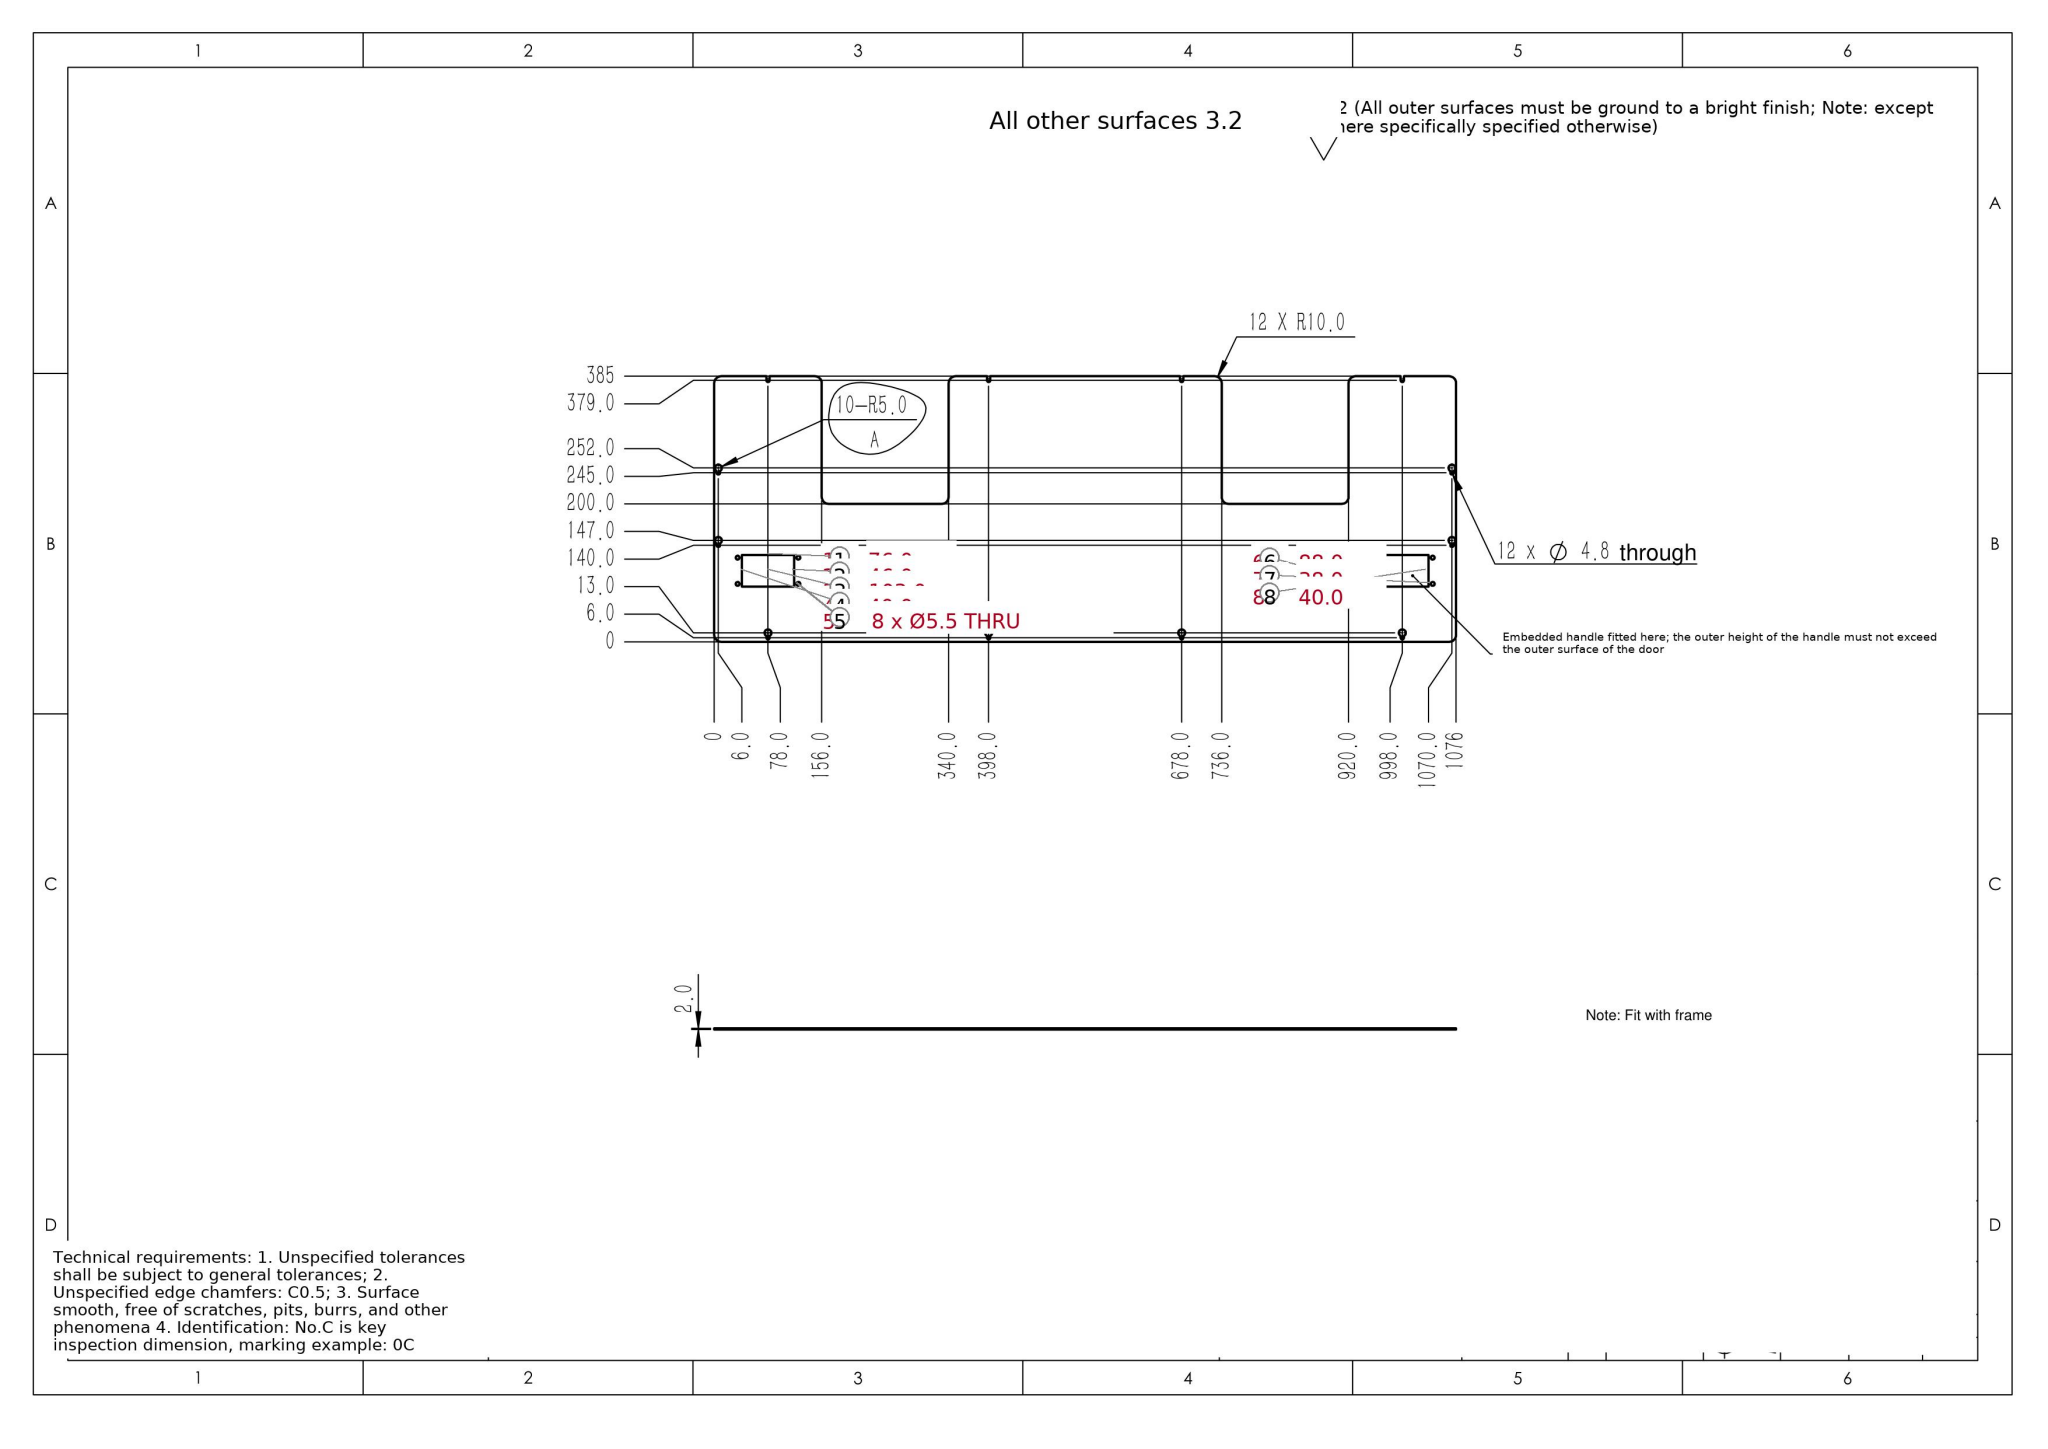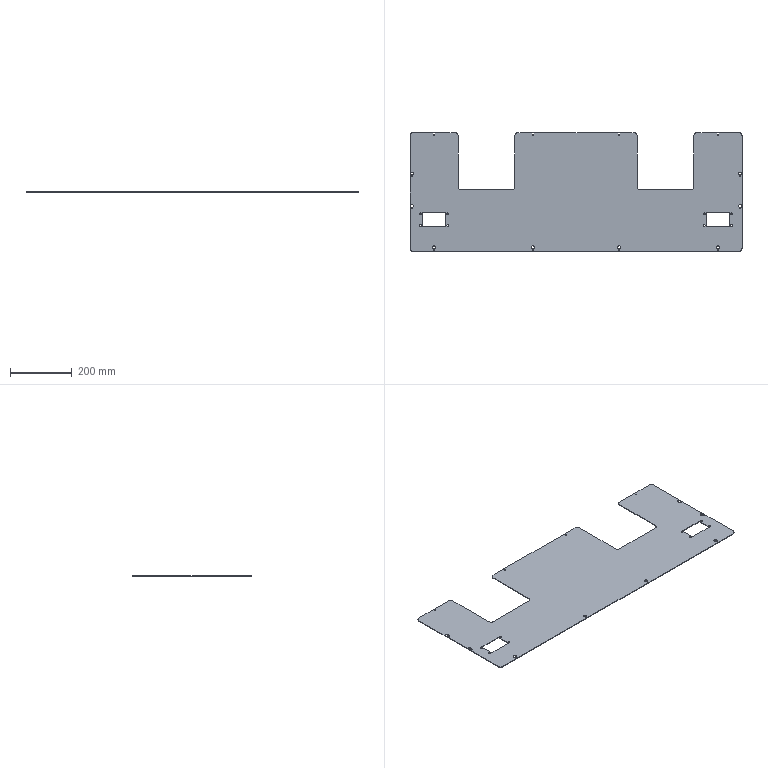Part | SolidWorks | mm | 1 solid | 114 faces | box 1076 x 385 x 2 mm | volume 675951 mm3 | cylinder 64 | plane 50 | commonest cylinder face diameters 10 x24 5.5 x16 20 x12 4.8 x12
build123d program:
from build123d import *

# Parameters (mm, degrees)
SKETCH1_W                      = 1076
SKETCH1_H                      = 385
BOSS_EXTRUDE1_DEPTH            = 2
SKETCH2_W                      = 184
SKETCH2_H                      = 185
CUT_EXTRUDE1_DEPTH             = 2
FILLET1_R                      = 10
F_4_8_4_8_DIAMETER_HOLE1_D     = 4.8
SKETCH5_W                      = 76
SKETCH5_H                      = 46
CUT_EXTRUDE2_DEPTH             = 10
F_5_5_5_5_DIAMETER_HOLE1_D     = 5.5
F_5_5_5_5_DIAMETER_HOLE1_DEPTH = 2
F_5_5_5_5_DIAMETER_HOLE1_TIP   = 1.652
CUT_EXTRUDE3_DEPTH             = 10
SKETCH11_W                     = 4.8
SKETCH11_H                     = 6
CUT_EXTRUDE4_DEPTH             = 10


with BuildPart() as part:
    # Sketch1 → Boss-Extrude1 (new body)
    with BuildSketch(Plane.XY):
        Rectangle(SKETCH1_W, SKETCH1_H)
    extrude(amount=BOSS_EXTRUDE1_DEPTH)

    # Sketch2 → Cut-Extrude1 (cut)
    with BuildSketch(Plane.XY.offset(2)):
        with Locations((-290, 100)):
            Rectangle(SKETCH2_W, SKETCH2_H)
        with Locations((290, 100)):
            Rectangle(SKETCH2_W, SKETCH2_H)
    extrude(amount=-CUT_EXTRUDE1_DEPTH, mode=Mode.SUBTRACT)

    # Fillet1
    fillet1_edges = [part.edges().sort_by_distance(p)[0] for p in [
        (-382, 7.5, 1),
        (-382, 192.5, 1),
        (-198, 192.5, 1),
        (-198, 7.5, 1),
        (198, 7.5, 1),
        (198, 192.5, 1),
        (382, 192.5, 1),
        (382, 7.5, 1),
        (538, -192.5, 1),
        (-538, -192.5, 1),
        (-538, 192.5, 1),
        (538, 192.5, 1),
    ]]
    fillet(fillet1_edges, radius=FILLET1_R)

    # 4.8 _4.8_ Diameter Hole1 (through all)
    with Locations(Plane(origin=(0, 0, 0), x_dir=(-1, 0, 0), z_dir=(0, 0, -1))):
        with Locations((-140, 186.5), (140, 186.5), (460, 186.5), (-460, 186.5), (-532, 52.5), (532, 52.5), (532, -52.5), (460, -186.5), (140, -186.5), (-140, -186.5), (-460, -186.5), (-532, -52.5)):
            Hole(F_4_8_4_8_DIAMETER_HOLE1_D / 2)

    # Sketch5 → Cut-Extrude2 (cut)
    with BuildSketch(Plane(origin=(0, 0, 0), x_dir=(-1, 0, 0), z_dir=(0, 0, -1))):
        with Locations((-460, -89.5)):
            Rectangle(SKETCH5_W, SKETCH5_H)
        with Locations((460, -89.5)):
            Rectangle(SKETCH5_W, SKETCH5_H)
    extrude(amount=-CUT_EXTRUDE2_DEPTH, mode=Mode.SUBTRACT)

    # 5.5 _5.5_ Diameter Hole1
    with Locations(Plane(origin=(0, 0, 0), x_dir=(-1, 0, 0), z_dir=(0, 0, -1))):
        with Locations((504, -108.5), (416, -108.5), (504, -70.5), (416, -70.5), (-416, -70.5), (-416, -108.5), (-504, -70.5), (-504, -108.5)):
            Hole(F_5_5_5_5_DIAMETER_HOLE1_D / 2, depth=F_5_5_5_5_DIAMETER_HOLE1_DEPTH)
            with Locations((0, 0, -(F_5_5_5_5_DIAMETER_HOLE1_DEPTH + F_5_5_5_5_DIAMETER_HOLE1_TIP / 2))):  # 118° drill point
                Cone(0, F_5_5_5_5_DIAMETER_HOLE1_D / 2, F_5_5_5_5_DIAMETER_HOLE1_TIP, mode=Mode.SUBTRACT)

    # Sketch10 → Cut-Extrude3 (cut)
    with BuildSketch(Plane.XY.offset(2)):
        with BuildLine():
            Line((462.4, -186.5), (462.4, -183.886))
            ThreePointArc((462.4, -183.886), (460, -174.5), (457.6, -183.886))
            Line((457.6, -183.886), (457.6, -186.5))
            Line((457.6, -186.5), (462.4, -186.5))
        make_face()
        with BuildLine():
            Line((142.4, -186.5), (137.6, -186.5))
            Line((137.6, -186.5), (137.6, -183.886))
            ThreePointArc((137.6, -183.886), (140, -174.5), (142.4, -183.886))
            Line((142.4, -183.886), (142.4, -186.5))
        make_face()
        with BuildLine():
            Line((-142.4, -186.5), (-142.4, -183.886))
            ThreePointArc((-142.4, -183.886), (-140, -174.5), (-137.6, -183.886))
            Line((-137.6, -183.886), (-137.6, -186.5))
            Line((-137.6, -186.5), (-142.4, -186.5))
        make_face()
        with BuildLine():
            Line((-457.6, -186.5), (-462.4, -186.5))
            Line((-462.4, -186.5), (-462.4, -183.886))
            ThreePointArc((-462.4, -183.886), (-460, -174.5), (-457.6, -183.886))
            Line((-457.6, -183.886), (-457.6, -186.5))
        make_face()
        with BuildLine():
            Line((534.4, -52.5), (529.6, -52.5))
            Line((529.6, -52.5), (529.6, -49.886))
            ThreePointArc((529.6, -49.886), (532, -40.5), (534.4, -49.886))
            Line((534.4, -49.886), (534.4, -52.5))
        make_face()
        with BuildLine():
            Line((534.4, 52.5), (529.6, 52.5))
            Line((529.6, 52.5), (529.6, 55.114))
            ThreePointArc((529.6, 55.114), (532, 64.5), (534.4, 55.114))
            Line((534.4, 55.114), (534.4, 52.5))
        make_face()
        with BuildLine():
            Line((-529.6, -52.5), (-534.4, -52.5))
            Line((-534.4, -52.5), (-534.4, -49.886))
            ThreePointArc((-534.4, -49.886), (-532, -40.5), (-529.6, -49.886))
            Line((-529.6, -49.886), (-529.6, -52.5))
        make_face()
        with BuildLine():
            Line((-529.6, 52.5), (-534.4, 52.5))
            Line((-534.4, 52.5), (-534.4, 55.114))
            ThreePointArc((-534.4, 55.114), (-532, 64.5), (-529.6, 55.114))
            Line((-529.6, 55.114), (-529.6, 52.5))
        make_face()
    extrude(amount=-CUT_EXTRUDE3_DEPTH, mode=Mode.SUBTRACT)

    # Sketch11 → Cut-Extrude4 (cut)
    with BuildSketch(Plane.XY.offset(2)):
        with Locations((460, 189.5)):
            Rectangle(SKETCH11_W, SKETCH11_H)
        with Locations((140, 189.5)):
            Rectangle(SKETCH11_W, SKETCH11_H)
        with Locations((-140, 189.5)):
            Rectangle(SKETCH11_W, SKETCH11_H)
        with Locations((-460, 189.5)):
            Rectangle(SKETCH11_W, SKETCH11_H)
    extrude(amount=-CUT_EXTRUDE4_DEPTH, mode=Mode.SUBTRACT)


solid = part.part